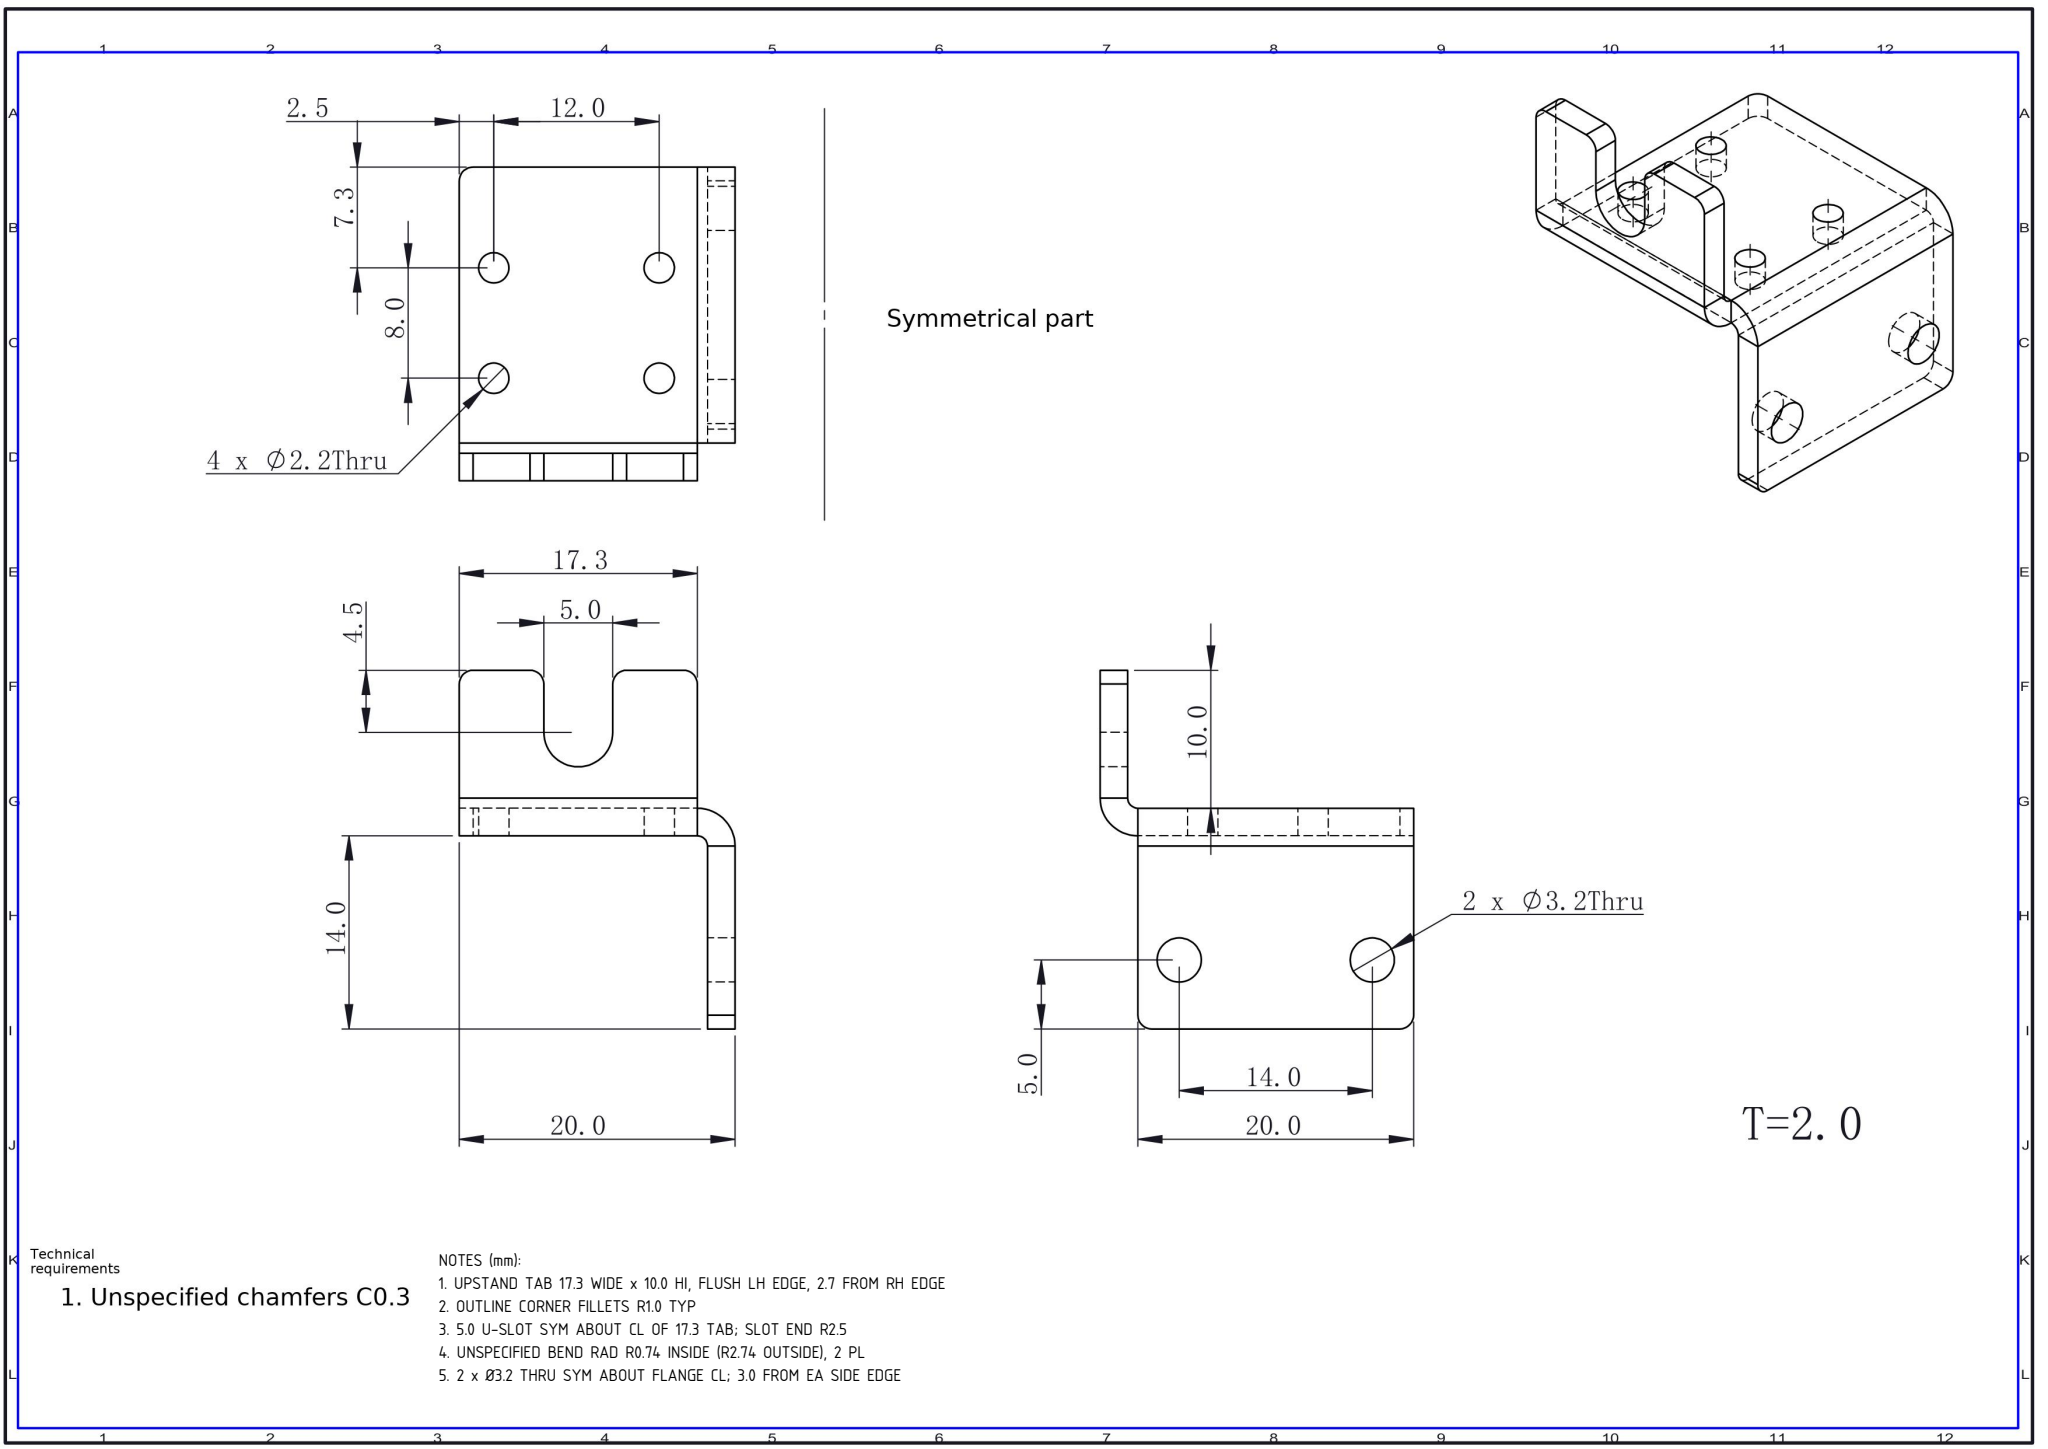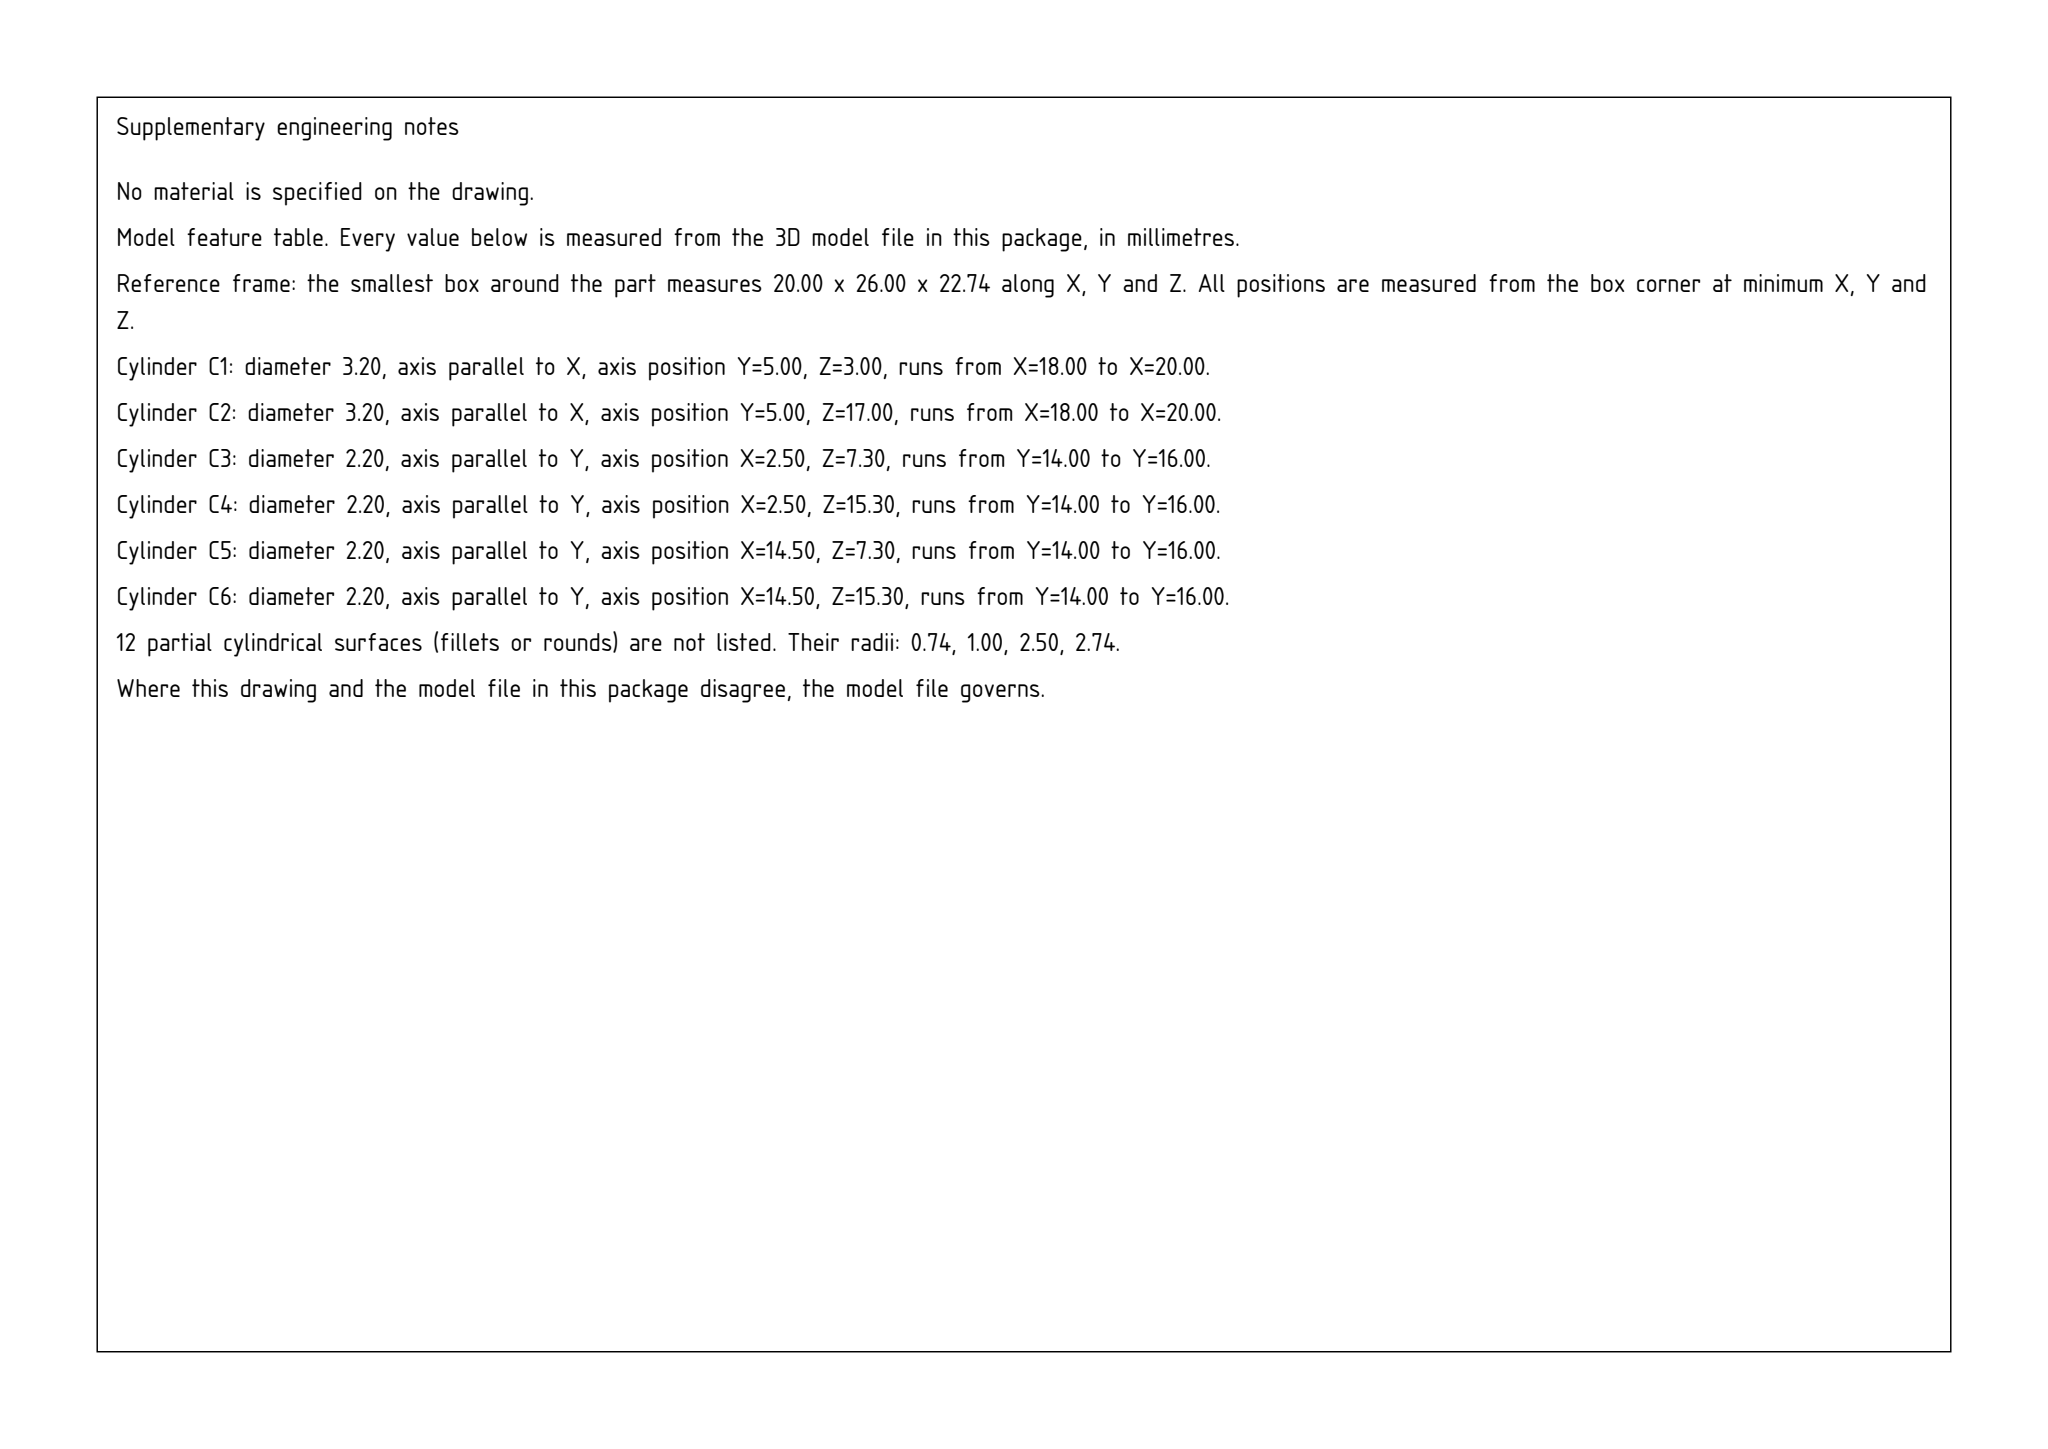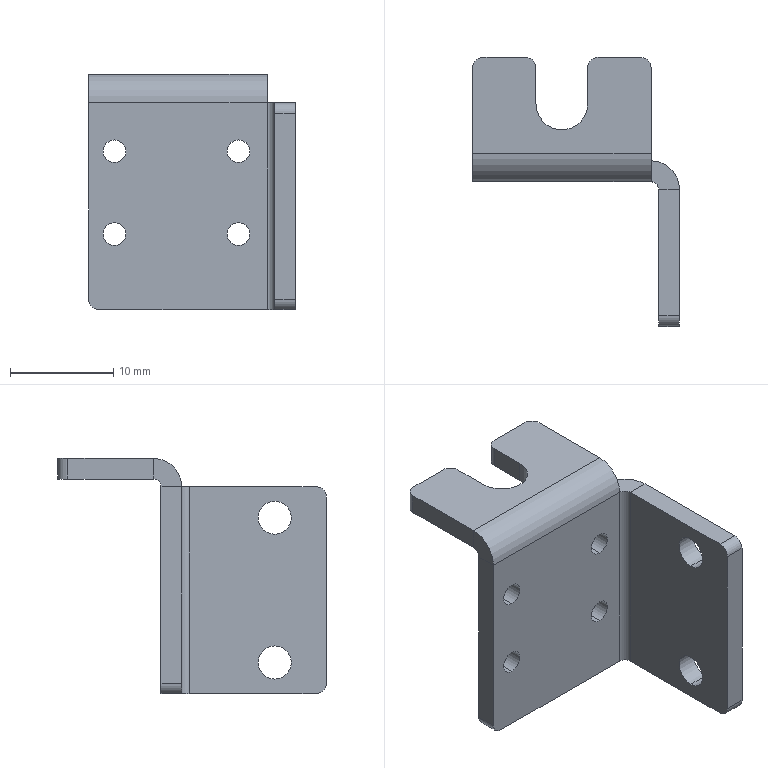Part | SolidWorks | mm | 1 solid | 45 faces | box 20 x 26 x 22.74 mm | volume 1614 mm3 | cylinder 24 | plane 21 | commonest cylinder face diameters 2.2 x8 2 x7 3.2 x4 5.473 x2 1.473 x2 5 x1
Drawing notes:
UPSTAND TAB 17.3 WIDE x 10.0 HI, FLUSH LH EDGE, 2.7 FROM RH EDGE | from the solid: Tab plate z20.74-22.74 spans x0-17.26 of 20.0 plate; y16.0-26.0 = 10.0 high
OUTLINE CORNER FILLETS R1.0 TYP | from the solid: Dia 2.0 cyls L2.0: axis x (1.0,1.0)&(1.0,19.0); axis y (1.0,1.0); axis z (1.0,25.0),(5.13,25.0),(12.13,25.0),(16.26,25.0)
5.0 U-SLOT SYM ABOUT CL OF 17.3 TAB; SLOT END R2.5 | from the solid: Slot sides x=6.13/11.13 (CL x=8.63=17.26/2); dia 5.0 cyl axis z @ (8.63,21.5) = R2.5 end, depth to y26 = 4.5
UNSPECIFIED BEND RAD R0.74 INSIDE (R2.74 OUTSIDE), 2 PL | from the solid: Bend cyls dia 1.473 & 5.473 (axis x @ y16.74,z20.0 L17.26; axis z @ x17.26,y13.26 L20.0) -> IR0.7365, OR2.736, T=2.0
2 x Ø3.2 THRU SYM ABOUT FLANGE CL; 3.0 FROM EA SIDE EDGE | from the solid: Flange width 20.0 with 14.0 hole spacing centered: (20.0-14.0)/2 = 3.0 from each edge, pair symmetric about flange centerline